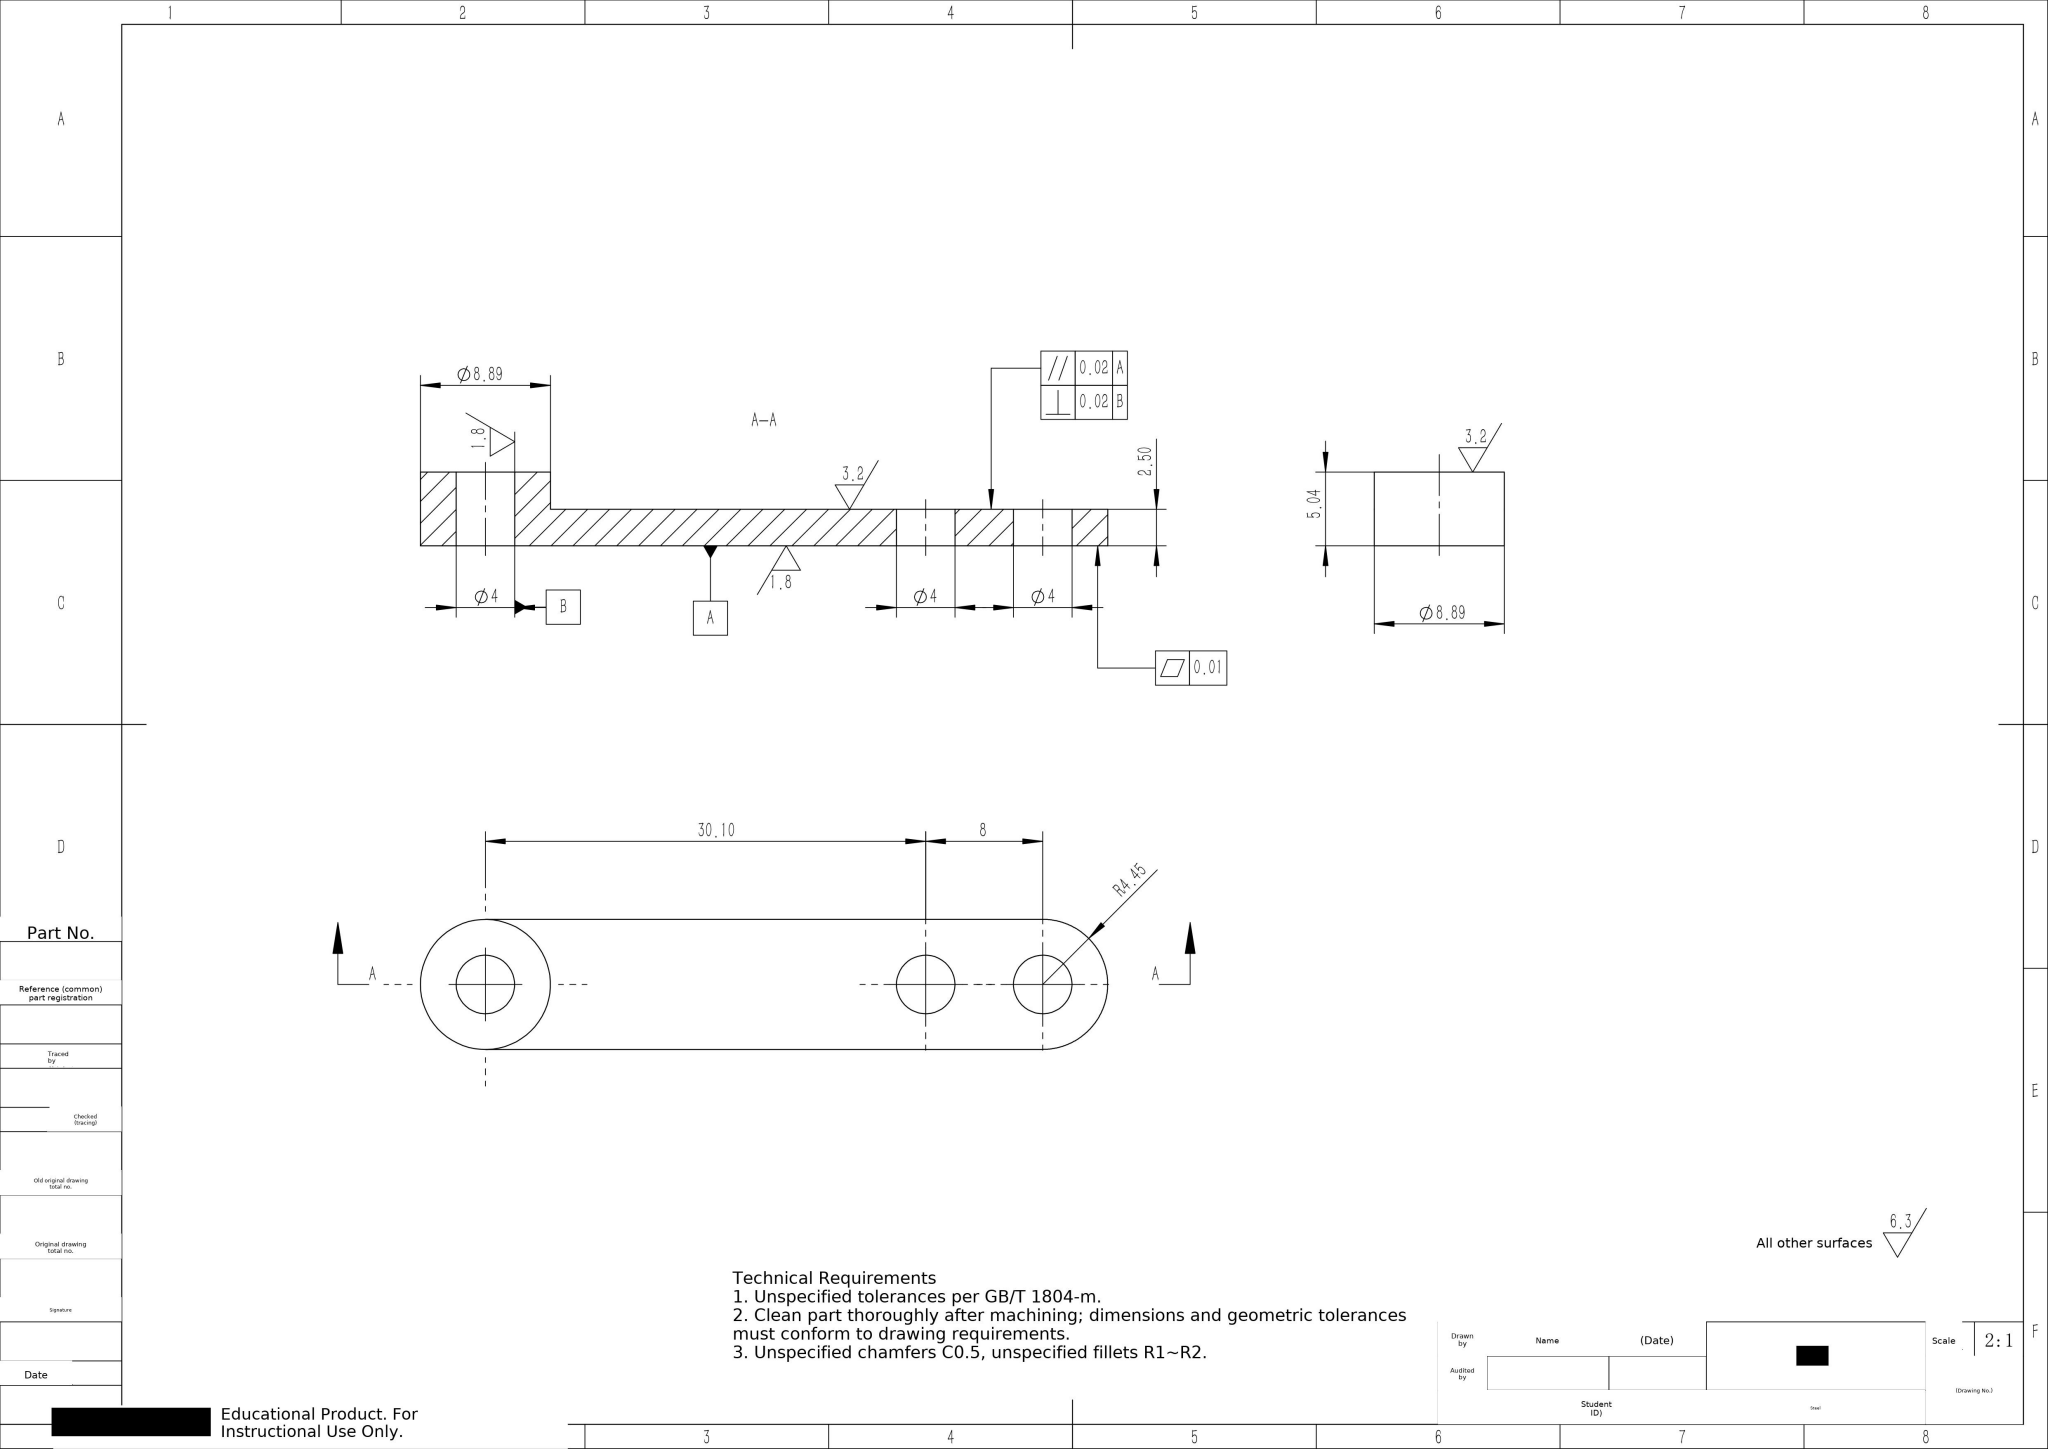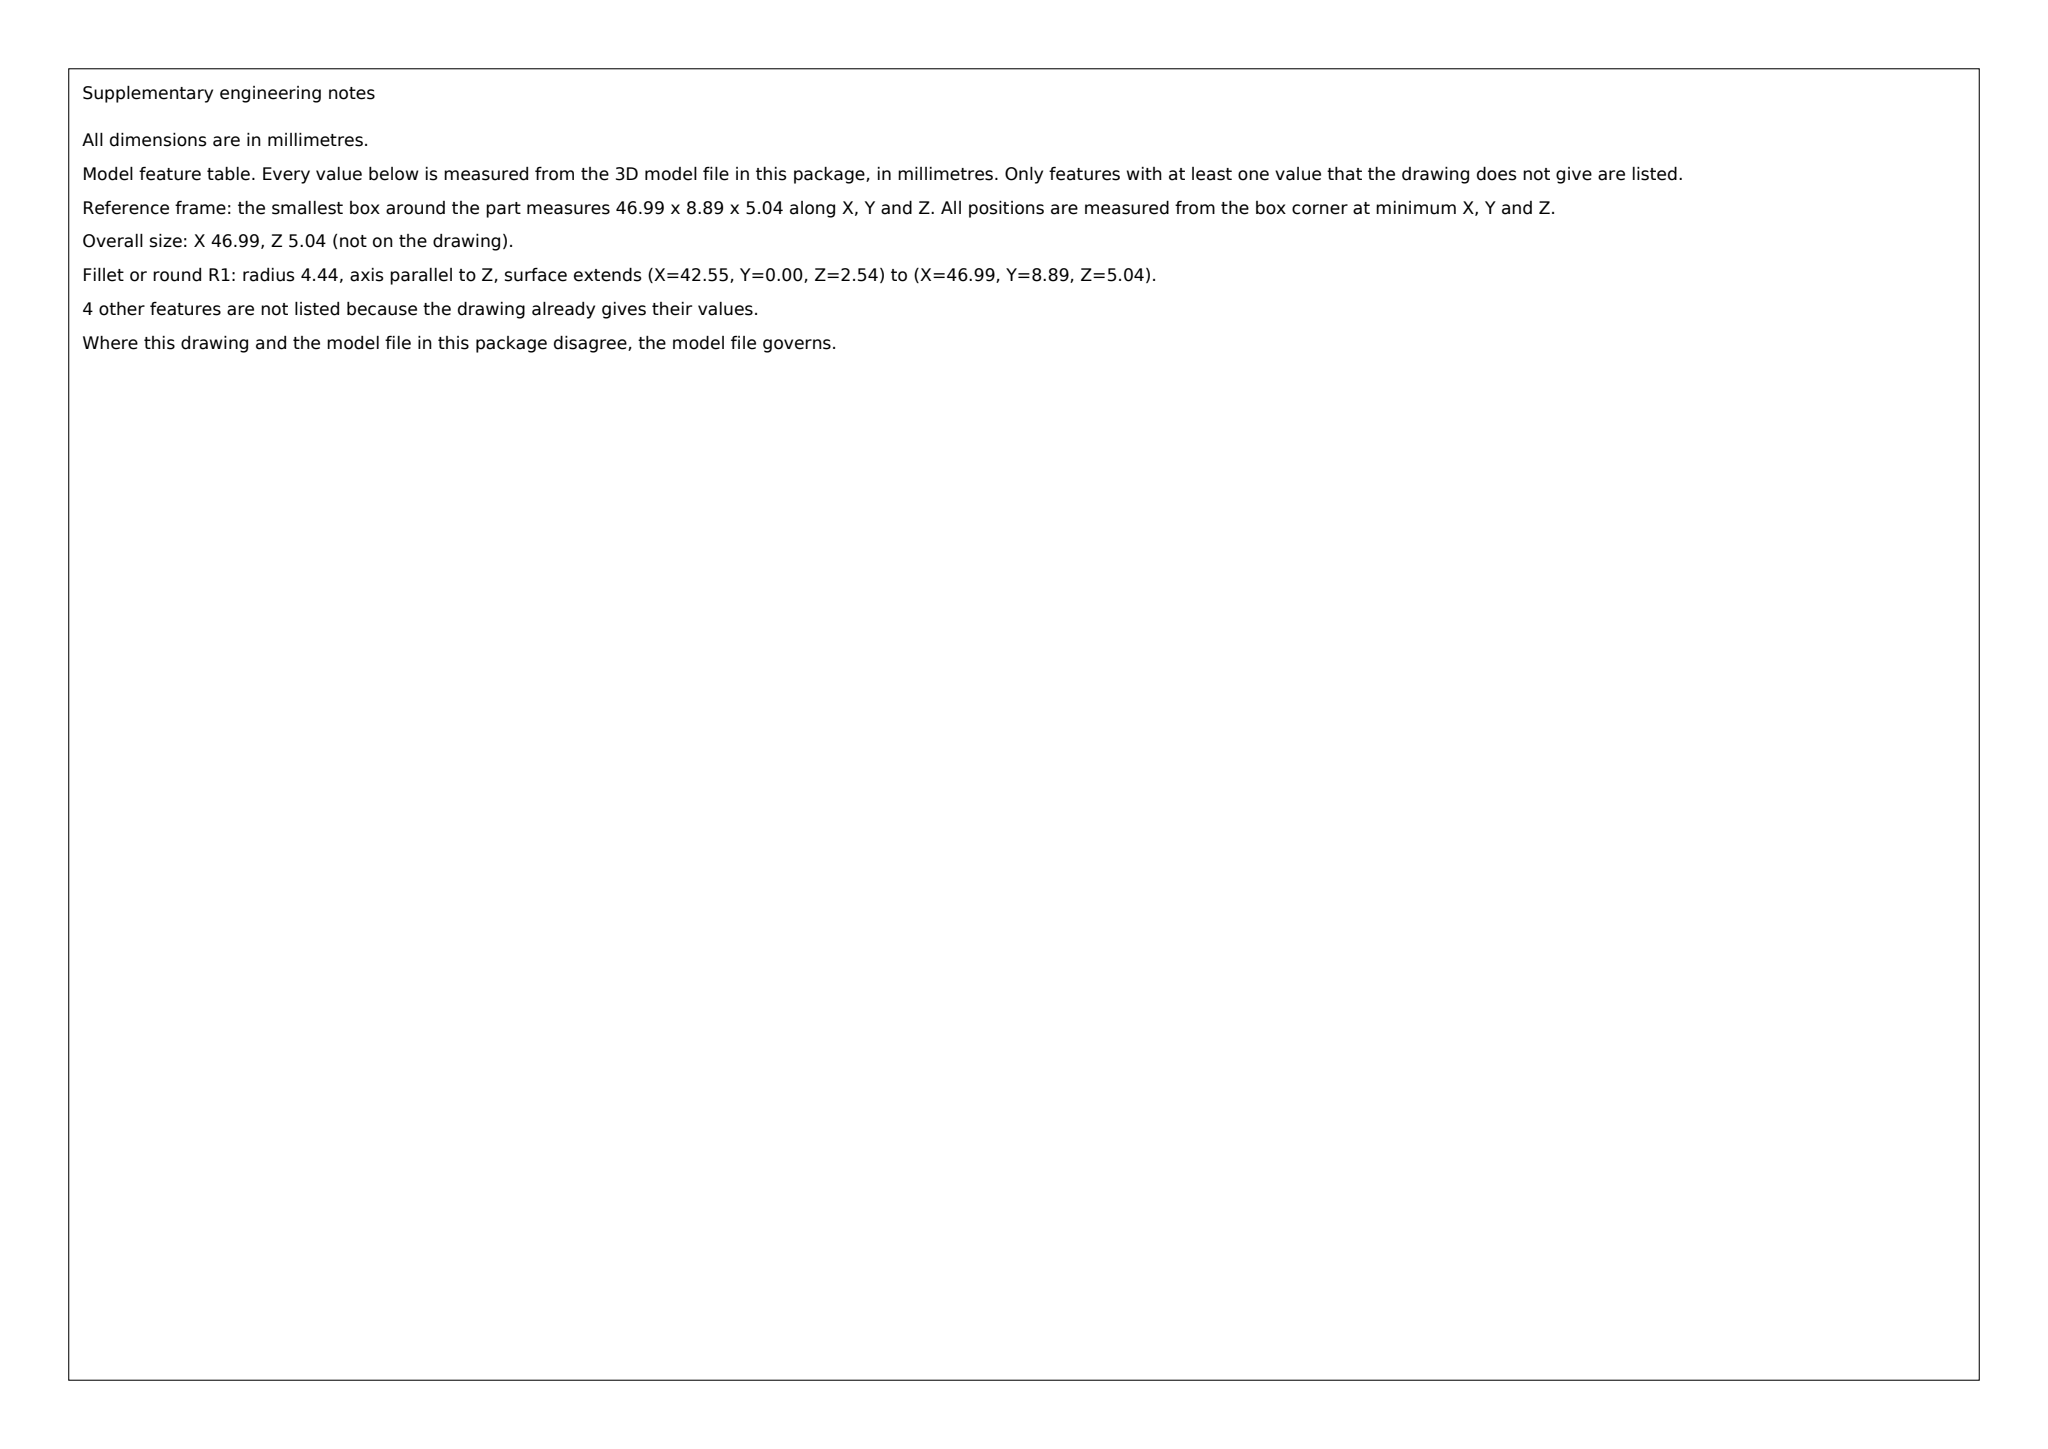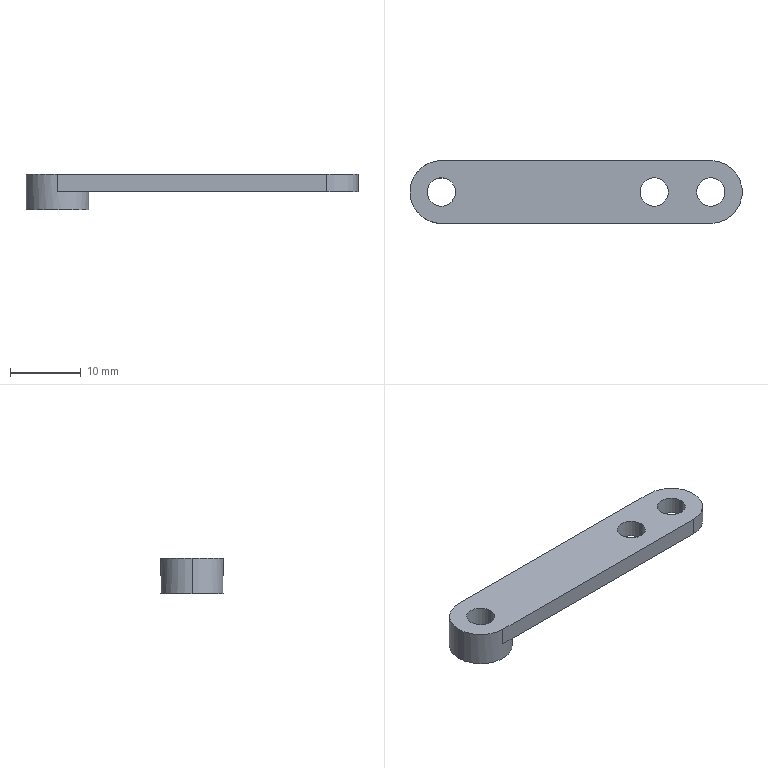Part | SolidWorks | mm | material Steel | 1 solid | 14 faces | box 46.99 x 8.89 x 5.04 mm | volume 1033 mm3 | cylinder 9 | plane 5 | commonest cylinder face diameters 4 x6 8.89 x3
build123d program:
from build123d import *

# Parameters (mm, degrees)
EXTRUDE1_DEPTH        = 2.5
SKETCH2_R             = 2
SKETCH2_R_2           = 1.5
CUT_EXTRUDE3_DEPTH    = 75.794
EXTRUDE2_START        = 2.54
SKETCH3_R             = 4.445
SKETCH3_R_2           = 1.587
EXTRUDE2_DEPTH        = 2.54
CROQUIS2_R            = 2
CORTAR_EXTRUIR2_DEPTH = 10


with BuildPart() as part:
    # Sketch1 → Extrude1 (new body)
    with BuildSketch(Plane.XY):
        with BuildLine():
            Line((-31.75, -8.255), (-69.85, -8.255))
            ThreePointArc((-69.85, -8.255), (-74.295, -3.81), (-69.85, 0.635))
            Line((-69.85, 0.635), (-31.75, 0.635))
            ThreePointArc((-31.75, 0.635), (-27.305, -3.81), (-31.75, -8.255))
        make_face()
    extrude(amount=EXTRUDE1_DEPTH)

    # Sketch2 → Cut-Extrude3 (cut, through all)
    with BuildSketch(Plane.XY):
        with Locations((-31.75, -3.81)):
            Circle(SKETCH2_R)
        with Locations((-39.75, -3.81)):
            Circle(SKETCH2_R)
        with Locations((-69.85, -3.81)):
            Circle(SKETCH2_R_2)
    extrude(amount=CUT_EXTRUDE3_DEPTH, mode=Mode.SUBTRACT)

    # Sketch3 → Extrude2 (add)
    with BuildSketch(Plane(origin=(0, 0, 0), x_dir=(-1, 0, 0), z_dir=(0, 0, -1)).offset(EXTRUDE2_START)):
        with Locations((69.85, -3.81)):
            Circle(SKETCH3_R)
        with Locations((69.85, -3.81)):
            Circle(SKETCH3_R_2, mode=Mode.SUBTRACT)
    extrude(amount=-EXTRUDE2_DEPTH)

    # Croquis2 → Cortar-Extruir2 (cut)
    with BuildSketch(Plane(origin=(0, 0, -2.54), x_dir=(-1, 0, 0), z_dir=(0, 0, -1))):
        with Locations((69.85, -3.81)):
            Circle(CROQUIS2_R)
    extrude(amount=-CORTAR_EXTRUIR2_DEPTH, mode=Mode.SUBTRACT)


solid = part.part
STEP:
#1=CARTESIAN_POINT('',(-71.85,-3.81,2.5));
#2=VERTEX_POINT('',#1);
#3=CARTESIAN_POINT('',(-67.85,-3.81,2.5));
#4=VERTEX_POINT('',#3);
#5=CARTESIAN_POINT('',(-69.85,-3.81,2.5));
#6=DIRECTION('',(0.,0.,1.));
#7=DIRECTION('',(1.,0.,0.));
#8=AXIS2_PLACEMENT_3D('',#5,#6,#7);
#9=CIRCLE('',#8,2.);
#10=EDGE_CURVE('',#2,#4,#9,.T.);
#11=ORIENTED_EDGE('',*,*,#10,.T.);
#12=CARTESIAN_POINT('',(-67.85,-3.81,-2.54));
#13=VERTEX_POINT('',#12);
#14=CARTESIAN_POINT('',(-67.85,-3.81,7.46));
#15=DIRECTION('',(0.,0.,-1.));
#16=VECTOR('',#15,1000.);
#17=LINE('',#14,#16);
#18=EDGE_CURVE('',#4,#13,#17,.T.);
#19=ORIENTED_EDGE('',*,*,#18,.T.);
#20=CARTESIAN_POINT('',(-71.85,-3.81,-2.54));
#21=VERTEX_POINT('',#20);
#22=CARTESIAN_POINT('',(-69.85,-3.81,-2.54));
#23=DIRECTION('',(0.,0.,-1.));
#24=DIRECTION('',(-1.,0.,0.));
#25=AXIS2_PLACEMENT_3D('',#22,#23,#24);
#26=CIRCLE('',#25,2.);
#27=EDGE_CURVE('',#13,#21,#26,.T.);
#28=ORIENTED_EDGE('',*,*,#27,.T.);
#29=CARTESIAN_POINT('',(-71.85,-3.81,7.46));
#30=DIRECTION('',(0.,0.,-1.));
#31=VECTOR('',#30,1000.);
#32=LINE('',#29,#31);
#33=EDGE_CURVE('',#2,#21,#32,.T.);
#34=ORIENTED_EDGE('',*,*,#33,.F.);
#35=EDGE_LOOP('',(#11,#19,#28,#34));
#36=FACE_OUTER_BOUND('',#35,.T.);
#37=CARTESIAN_POINT('',(-69.85,-3.81,7.46));
#38=DIRECTION('',(0.,0.,-1.));
#39=DIRECTION('',(-1.,0.,0.));
#40=AXIS2_PLACEMENT_3D('',#37,#38,#39);
#41=CYLINDRICAL_SURFACE('',#40,2.);
#42=ADVANCED_FACE('',(#36),#41,.F.);
#43=CARTESIAN_POINT('',(-41.75,-3.81,2.5));
#44=VERTEX_POINT('',#43);
#45=CARTESIAN_POINT('',(-37.75,-3.81,2.5));
#46=VERTEX_POINT('',#45);
#47=CARTESIAN_POINT('',(-39.75,-3.81,2.5));
#48=DIRECTION('',(0.,0.,1.));
#49=DIRECTION('',(1.,0.,0.));
#50=AXIS2_PLACEMENT_3D('',#47,#48,#49);
#51=CIRCLE('',#50,2.);
#52=EDGE_CURVE('',#44,#46,#51,.T.);
#53=ORIENTED_EDGE('',*,*,#52,.T.);
#54=CARTESIAN_POINT('',(-37.75,-3.81,0.));
#55=VERTEX_POINT('',#54);
#56=CARTESIAN_POINT('',(-37.75,-3.81,2.5));
#57=DIRECTION('',(0.,0.,-1.));
#58=VECTOR('',#57,1000.);
#59=LINE('',#56,#58);
#60=EDGE_CURVE('',#46,#55,#59,.T.);
#61=ORIENTED_EDGE('',*,*,#60,.T.);
#62=CARTESIAN_POINT('',(-41.75,-3.81,0.));
#63=VERTEX_POINT('',#62);
#64=CARTESIAN_POINT('',(-39.75,-3.81,0.));
#65=DIRECTION('',(0.,0.,1.));
#66=DIRECTION('',(1.,0.,0.));
#67=AXIS2_PLACEMENT_3D('',#64,#65,#66);
#68=CIRCLE('',#67,2.);
#69=EDGE_CURVE('',#63,#55,#68,.T.);
#70=ORIENTED_EDGE('',*,*,#69,.F.);
#71=CARTESIAN_POINT('',(-41.75,-3.81,2.5));
#72=DIRECTION('',(0.,0.,-1.));
#73=VECTOR('',#72,1000.);
#74=LINE('',#71,#73);
#75=EDGE_CURVE('',#44,#63,#74,.T.);
#76=ORIENTED_EDGE('',*,*,#75,.F.);
#77=EDGE_LOOP('',(#53,#61,#70,#76));
#78=FACE_OUTER_BOUND('',#77,.T.);
#79=CARTESIAN_POINT('',(-39.75,-3.81,2.5));
#80=DIRECTION('',(0.,0.,-1.));
#81=DIRECTION('',(-1.,0.,0.));
#82=AXIS2_PLACEMENT_3D('',#79,#80,#81);
#83=CYLINDRICAL_SURFACE('',#82,2.);
#84=ADVANCED_FACE('',(#78),#83,.F.);
#85=CARTESIAN_POINT('',(-33.75,-3.81,2.5));
#86=VERTEX_POINT('',#85);
#87=CARTESIAN_POINT('',(-29.75,-3.81,2.5));
#88=VERTEX_POINT('',#87);
#89=CARTESIAN_POINT('',(-31.75,-3.81,2.5));
#90=DIRECTION('',(0.,0.,1.));
#91=DIRECTION('',(1.,0.,0.));
#92=AXIS2_PLACEMENT_3D('',#89,#90,#91);
#93=CIRCLE('',#92,2.);
#94=EDGE_CURVE('',#86,#88,#93,.T.);
#95=ORIENTED_EDGE('',*,*,#94,.T.);
#96=CARTESIAN_POINT('',(-29.75,-3.81,0.));
#97=VERTEX_POINT('',#96);
#98=CARTESIAN_POINT('',(-29.75,-3.81,2.5));
#99=DIRECTION('',(0.,0.,-1.));
#100=VECTOR('',#99,1000.);
#101=LINE('',#98,#100);
#102=EDGE_CURVE('',#88,#97,#101,.T.);
#103=ORIENTED_EDGE('',*,*,#102,.T.);
#104=CARTESIAN_POINT('',(-33.75,-3.81,0.));
#105=VERTEX_POINT('',#104);
#106=CARTESIAN_POINT('',(-31.75,-3.81,0.));
#107=DIRECTION('',(0.,0.,1.));
#108=DIRECTION('',(1.,0.,0.));
#109=AXIS2_PLACEMENT_3D('',#106,#107,#108);
#110=CIRCLE('',#109,2.);
#111=EDGE_CURVE('',#105,#97,#110,.T.);
#112=ORIENTED_EDGE('',*,*,#111,.F.);
#113=CARTESIAN_POINT('',(-33.75,-3.81,2.5));
#114=DIRECTION('',(0.,0.,-1.));
#115=VECTOR('',#114,1000.);
#116=LINE('',#113,#115);
#117=EDGE_CURVE('',#86,#105,#116,.T.);
#118=ORIENTED_EDGE('',*,*,#117,.F.);
#119=EDGE_LOOP('',(#95,#103,#112,#118));
#120=FACE_OUTER_BOUND('',#119,.T.);
#121=CARTESIAN_POINT('',(-31.75,-3.81,2.5));
#122=DIRECTION('',(0.,0.,-1.));
#123=DIRECTION('',(-1.,0.,0.));
#124=AXIS2_PLACEMENT_3D('',#121,#122,#123);
#125=CYLINDRICAL_SURFACE('',#124,2.);
#126=ADVANCED_FACE('',(#120),#125,.F.);
#127=CARTESIAN_POINT('',(-69.85,0.635,0.));
#128=VERTEX_POINT('',#127);
#129=CARTESIAN_POINT('',(-65.405,-3.81,0.));
#130=VERTEX_POINT('',#129);
#131=CARTESIAN_POINT('',(-69.85,-3.81,0.));
#132=DIRECTION('',(0.,0.,-1.));
#133=DIRECTION('',(-1.,0.,0.));
#134=AXIS2_PLACEMENT_3D('',#131,#132,#133);
#135=CIRCLE('',#134,4.445);
#136=EDGE_CURVE('',#128,#130,#135,.T.);
#137=ORIENTED_EDGE('',*,*,#136,.T.);
#138=CARTESIAN_POINT('',(-65.405,-3.81,-2.54));
#139=VERTEX_POINT('',#138);
#140=CARTESIAN_POINT('',(-65.405,-3.81,2.5));
#141=DIRECTION('',(0.,0.,-1.));
#142=VECTOR('',#141,1000.);
#143=LINE('',#140,#142);
#144=EDGE_CURVE('',#130,#139,#143,.T.);
#145=ORIENTED_EDGE('',*,*,#144,.T.);
#146=CARTESIAN_POINT('',(-74.295,-3.81,-2.54));
#147=VERTEX_POINT('',#146);
#148=CARTESIAN_POINT('',(-69.85,-3.81,-2.54));
#149=DIRECTION('',(0.,0.,-1.));
#150=DIRECTION('',(-1.,0.,0.));
#151=AXIS2_PLACEMENT_3D('',#148,#149,#150);
#152=CIRCLE('',#151,4.445);
#153=EDGE_CURVE('',#147,#139,#152,.T.);
#154=ORIENTED_EDGE('',*,*,#153,.F.);
#155=CARTESIAN_POINT('',(-74.295,-3.81,2.5));
#156=VERTEX_POINT('',#155);
#157=CARTESIAN_POINT('',(-74.295,-3.81,2.5));
#158=DIRECTION('',(0.,0.,-1.));
#159=VECTOR('',#158,1000.);
#160=LINE('',#157,#159);
#161=EDGE_CURVE('',#156,#147,#160,.T.);
#162=ORIENTED_EDGE('',*,*,#161,.F.);
#163=CARTESIAN_POINT('',(-69.85,0.635,2.5));
#164=VERTEX_POINT('',#163);
#165=CARTESIAN_POINT('',(-69.85,-3.81,2.5));
#166=DIRECTION('',(0.,0.,1.));
#167=DIRECTION('',(1.,0.,0.));
#168=AXIS2_PLACEMENT_3D('',#165,#166,#167);
#169=CIRCLE('',#168,4.445);
#170=EDGE_CURVE('',#164,#156,#169,.T.);
#171=ORIENTED_EDGE('',*,*,#170,.F.);
#172=CARTESIAN_POINT('',(-69.85,0.635,2.5));
#173=DIRECTION('',(0.,0.,-1.));
#174=VECTOR('',#173,1000.);
#175=LINE('',#172,#174);
#176=EDGE_CURVE('',#164,#128,#175,.T.);
#177=ORIENTED_EDGE('',*,*,#176,.T.);
#178=EDGE_LOOP('',(#137,#145,#154,#162,#171,#177));
#179=FACE_OUTER_BOUND('',#178,.T.);
#180=CARTESIAN_POINT('',(-69.85,-3.81,2.5));
#181=DIRECTION('',(0.,0.,-1.));
#182=DIRECTION('',(-1.,0.,0.));
#183=AXIS2_PLACEMENT_3D('',#180,#181,#182);
#184=CYLINDRICAL_SURFACE('',#183,4.445);
#185=ADVANCED_FACE('',(#179),#184,.T.);
#186=ORIENTED_EDGE('',*,*,#111,.T.);
#187=CARTESIAN_POINT('',(-31.75,-3.81,0.));
#188=DIRECTION('',(0.,0.,1.));
#189=DIRECTION('',(1.,0.,0.));
#190=AXIS2_PLACEMENT_3D('',#187,#188,#189);
#191=CIRCLE('',#190,2.);
#192=EDGE_CURVE('',#97,#105,#191,.T.);
#193=ORIENTED_EDGE('',*,*,#192,.T.);
#194=EDGE_LOOP('',(#186,#193));
#195=FACE_BOUND('',#194,.T.);
#196=ORIENTED_EDGE('',*,*,#69,.T.);
#197=CARTESIAN_POINT('',(-39.75,-3.81,0.));
#198=DIRECTION('',(0.,0.,1.));
#199=DIRECTION('',(1.,0.,0.));
#200=AXIS2_PLACEMENT_3D('',#197,#198,#199);
#201=CIRCLE('',#200,2.);
#202=EDGE_CURVE('',#55,#63,#201,.T.);
#203=ORIENTED_EDGE('',*,*,#202,.T.);
#204=EDGE_LOOP('',(#196,#203));
#205=FACE_BOUND('',#204,.T.);
#206=ORIENTED_EDGE('',*,*,#136,.F.);
#207=CARTESIAN_POINT('',(-31.75,0.635,0.));
#208=VERTEX_POINT('',#207);
#209=CARTESIAN_POINT('',(-31.75,0.635,0.));
#210=DIRECTION('',(-1.,0.,0.));
#211=VECTOR('',#210,1000.);
#212=LINE('',#209,#211);
#213=EDGE_CURVE('',#208,#128,#212,.T.);
#214=ORIENTED_EDGE('',*,*,#213,.F.);
#215=CARTESIAN_POINT('',(-31.75,-8.255,0.));
#216=VERTEX_POINT('',#215);
#217=CARTESIAN_POINT('',(-31.75,-3.81,0.));
#218=DIRECTION('',(0.,0.,1.));
#219=DIRECTION('',(1.,0.,0.));
#220=AXIS2_PLACEMENT_3D('',#217,#218,#219);
#221=CIRCLE('',#220,4.445);
#222=EDGE_CURVE('',#216,#208,#221,.T.);
#223=ORIENTED_EDGE('',*,*,#222,.F.);
#224=CARTESIAN_POINT('',(-69.85,-8.255,0.));
#225=VERTEX_POINT('',#224);
#226=CARTESIAN_POINT('',(-31.75,-8.255,0.));
#227=DIRECTION('',(1.,0.,0.));
#228=VECTOR('',#227,1000.);
#229=LINE('',#226,#228);
#230=EDGE_CURVE('',#225,#216,#229,.T.);
#231=ORIENTED_EDGE('',*,*,#230,.F.);
#232=CARTESIAN_POINT('',(-69.85,-3.81,0.));
#233=DIRECTION('',(0.,0.,-1.));
#234=DIRECTION('',(-1.,0.,0.));
#235=AXIS2_PLACEMENT_3D('',#232,#233,#234);
#236=CIRCLE('',#235,4.445);
#237=EDGE_CURVE('',#130,#225,#236,.T.);
#238=ORIENTED_EDGE('',*,*,#237,.F.);
#239=EDGE_LOOP('',(#206,#214,#223,#231,#238));
#240=FACE_OUTER_BOUND('',#239,.T.);
#241=CARTESIAN_POINT('',(-31.75,-3.81,0.));
#242=DIRECTION('',(0.,0.,1.));
#243=DIRECTION('',(1.,0.,0.));
#244=AXIS2_PLACEMENT_3D('',#241,#242,#243);
#245=PLANE('',#244);
#246=ADVANCED_FACE('',(#195,#205,#240),#245,.F.);
#247=ORIENTED_EDGE('',*,*,#10,.F.);
#248=CARTESIAN_POINT('',(-69.85,-3.81,2.5));
#249=DIRECTION('',(0.,0.,1.));
#250=DIRECTION('',(1.,0.,0.));
#251=AXIS2_PLACEMENT_3D('',#248,#249,#250);
#252=CIRCLE('',#251,2.);
#253=EDGE_CURVE('',#4,#2,#252,.T.);
#254=ORIENTED_EDGE('',*,*,#253,.F.);
#255=EDGE_LOOP('',(#247,#254));
#256=FACE_BOUND('',#255,.T.);
#257=ORIENTED_EDGE('',*,*,#52,.F.);
#258=CARTESIAN_POINT('',(-39.75,-3.81,2.5));
#259=DIRECTION('',(0.,0.,1.));
#260=DIRECTION('',(1.,0.,0.));
#261=AXIS2_PLACEMENT_3D('',#258,#259,#260);
#262=CIRCLE('',#261,2.);
#263=EDGE_CURVE('',#46,#44,#262,.T.);
#264=ORIENTED_EDGE('',*,*,#263,.F.);
#265=EDGE_LOOP('',(#257,#264));
#266=FACE_BOUND('',#265,.T.);
#267=CARTESIAN_POINT('',(-31.75,-8.255,2.5));
#268=VERTEX_POINT('',#267);
#269=CARTESIAN_POINT('',(-31.75,0.635,2.5));
#270=VERTEX_POINT('',#269);
#271=CARTESIAN_POINT('',(-31.75,-3.81,2.5));
#272=DIRECTION('',(0.,0.,1.));
#273=DIRECTION('',(1.,0.,0.));
#274=AXIS2_PLACEMENT_3D('',#271,#272,#273);
#275=CIRCLE('',#274,4.445);
#276=EDGE_CURVE('',#268,#270,#275,.T.);
#277=ORIENTED_EDGE('',*,*,#276,.T.);
#278=CARTESIAN_POINT('',(-31.75,0.635,2.5));
#279=DIRECTION('',(-1.,0.,0.));
#280=VECTOR('',#279,1000.);
#281=LINE('',#278,#280);
#282=EDGE_CURVE('',#270,#164,#281,.T.);
#283=ORIENTED_EDGE('',*,*,#282,.T.);
#284=ORIENTED_EDGE('',*,*,#170,.T.);
#285=CARTESIAN_POINT('',(-69.85,-8.255,2.5));
#286=VERTEX_POINT('',#285);
#287=CARTESIAN_POINT('',(-69.85,-3.81,2.5));
#288=DIRECTION('',(0.,0.,1.));
#289=DIRECTION('',(1.,0.,0.));
#290=AXIS2_PLACEMENT_3D('',#287,#288,#289);
#291=CIRCLE('',#290,4.445);
#292=EDGE_CURVE('',#156,#286,#291,.T.);
#293=ORIENTED_EDGE('',*,*,#292,.T.);
#294=CARTESIAN_POINT('',(-31.75,-8.255,2.5));
#295=DIRECTION('',(1.,0.,0.));
#296=VECTOR('',#295,1000.);
#297=LINE('',#294,#296);
#298=EDGE_CURVE('',#286,#268,#297,.T.);
#299=ORIENTED_EDGE('',*,*,#298,.T.);
#300=EDGE_LOOP('',(#277,#283,#284,#293,#299));
#301=FACE_OUTER_BOUND('',#300,.T.);
#302=ORIENTED_EDGE('',*,*,#94,.F.);
#303=CARTESIAN_POINT('',(-31.75,-3.81,2.5));
#304=DIRECTION('',(0.,0.,1.));
#305=DIRECTION('',(1.,0.,0.));
#306=AXIS2_PLACEMENT_3D('',#303,#304,#305);
#307=CIRCLE('',#306,2.);
#308=EDGE_CURVE('',#88,#86,#307,.T.);
#309=ORIENTED_EDGE('',*,*,#308,.F.);
#310=EDGE_LOOP('',(#302,#309));
#311=FACE_BOUND('',#310,.T.);
#312=CARTESIAN_POINT('',(-31.75,-3.81,2.5));
#313=DIRECTION('',(0.,0.,1.));
#314=DIRECTION('',(1.,0.,0.));
#315=AXIS2_PLACEMENT_3D('',#312,#313,#314);
#316=PLANE('',#315);
#317=ADVANCED_FACE('',(#256,#266,#301,#311),#316,.T.);
#318=ORIENTED_EDGE('',*,*,#222,.T.);
#319=CARTESIAN_POINT('',(-31.75,0.635,2.5));
#320=DIRECTION('',(0.,0.,-1.));
#321=VECTOR('',#320,1000.);
#322=LINE('',#319,#321);
#323=EDGE_CURVE('',#270,#208,#322,.T.);
#324=ORIENTED_EDGE('',*,*,#323,.F.);
#325=ORIENTED_EDGE('',*,*,#276,.F.);
#326=CARTESIAN_POINT('',(-31.75,-8.255,2.5));
#327=DIRECTION('',(0.,0.,-1.));
#328=VECTOR('',#327,1000.);
#329=LINE('',#326,#328);
#330=EDGE_CURVE('',#268,#216,#329,.T.);
#331=ORIENTED_EDGE('',*,*,#330,.T.);
#332=EDGE_LOOP('',(#318,#324,#325,#331));
#333=FACE_OUTER_BOUND('',#332,.T.);
#334=CARTESIAN_POINT('',(-31.75,-3.81,2.5));
#335=DIRECTION('',(0.,0.,-1.));
#336=DIRECTION('',(-1.,0.,0.));
#337=AXIS2_PLACEMENT_3D('',#334,#335,#336);
#338=CYLINDRICAL_SURFACE('',#337,4.445);
#339=ADVANCED_FACE('',(#333),#338,.T.);
#340=ORIENTED_EDGE('',*,*,#213,.T.);
#341=ORIENTED_EDGE('',*,*,#176,.F.);
#342=ORIENTED_EDGE('',*,*,#282,.F.);
#343=ORIENTED_EDGE('',*,*,#323,.T.);
#344=EDGE_LOOP('',(#340,#341,#342,#343));
#345=FACE_OUTER_BOUND('',#344,.T.);
#346=CARTESIAN_POINT('',(-31.75,0.635,2.5));
#347=DIRECTION('',(0.,-1.,0.));
#348=DIRECTION('',(0.,0.,-1.));
#349=AXIS2_PLACEMENT_3D('',#346,#347,#348);
#350=PLANE('',#349);
#351=ADVANCED_FACE('',(#345),#350,.F.);
#352=ORIENTED_EDGE('',*,*,#144,.F.);
#353=ORIENTED_EDGE('',*,*,#237,.T.);
#354=CARTESIAN_POINT('',(-69.85,-8.255,2.5));
#355=DIRECTION('',(0.,0.,-1.));
#356=VECTOR('',#355,1000.);
#357=LINE('',#354,#356);
#358=EDGE_CURVE('',#286,#225,#357,.T.);
#359=ORIENTED_EDGE('',*,*,#358,.F.);
#360=ORIENTED_EDGE('',*,*,#292,.F.);
#361=ORIENTED_EDGE('',*,*,#161,.T.);
#362=CARTESIAN_POINT('',(-69.85,-3.81,-2.54));
#363=DIRECTION('',(0.,0.,-1.));
#364=DIRECTION('',(-1.,0.,0.));
#365=AXIS2_PLACEMENT_3D('',#362,#363,#364);
#366=CIRCLE('',#365,4.445);
#367=EDGE_CURVE('',#139,#147,#366,.T.);
#368=ORIENTED_EDGE('',*,*,#367,.F.);
#369=EDGE_LOOP('',(#352,#353,#359,#360,#361,#368));
#370=FACE_OUTER_BOUND('',#369,.T.);
#371=CARTESIAN_POINT('',(-69.85,-3.81,2.5));
#372=DIRECTION('',(0.,0.,-1.));
#373=DIRECTION('',(-1.,0.,0.));
#374=AXIS2_PLACEMENT_3D('',#371,#372,#373);
#375=CYLINDRICAL_SURFACE('',#374,4.445);
#376=ADVANCED_FACE('',(#370),#375,.T.);
#377=ORIENTED_EDGE('',*,*,#230,.T.);
#378=ORIENTED_EDGE('',*,*,#330,.F.);
#379=ORIENTED_EDGE('',*,*,#298,.F.);
#380=ORIENTED_EDGE('',*,*,#358,.T.);
#381=EDGE_LOOP('',(#377,#378,#379,#380));
#382=FACE_OUTER_BOUND('',#381,.T.);
#383=CARTESIAN_POINT('',(-31.75,-8.255,2.5));
#384=DIRECTION('',(0.,1.,0.));
#385=DIRECTION('',(0.,0.,1.));
#386=AXIS2_PLACEMENT_3D('',#383,#384,#385);
#387=PLANE('',#386);
#388=ADVANCED_FACE('',(#382),#387,.F.);
#389=ORIENTED_EDGE('',*,*,#102,.F.);
#390=ORIENTED_EDGE('',*,*,#308,.T.);
#391=ORIENTED_EDGE('',*,*,#117,.T.);
#392=ORIENTED_EDGE('',*,*,#192,.F.);
#393=EDGE_LOOP('',(#389,#390,#391,#392));
#394=FACE_OUTER_BOUND('',#393,.T.);
#395=CARTESIAN_POINT('',(-31.75,-3.81,2.5));
#396=DIRECTION('',(0.,0.,-1.));
#397=DIRECTION('',(-1.,0.,0.));
#398=AXIS2_PLACEMENT_3D('',#395,#396,#397);
#399=CYLINDRICAL_SURFACE('',#398,2.);
#400=ADVANCED_FACE('',(#394),#399,.F.);
#401=ORIENTED_EDGE('',*,*,#60,.F.);
#402=ORIENTED_EDGE('',*,*,#263,.T.);
#403=ORIENTED_EDGE('',*,*,#75,.T.);
#404=ORIENTED_EDGE('',*,*,#202,.F.);
#405=EDGE_LOOP('',(#401,#402,#403,#404));
#406=FACE_OUTER_BOUND('',#405,.T.);
#407=CARTESIAN_POINT('',(-39.75,-3.81,2.5));
#408=DIRECTION('',(0.,0.,-1.));
#409=DIRECTION('',(-1.,0.,0.));
#410=AXIS2_PLACEMENT_3D('',#407,#408,#409);
#411=CYLINDRICAL_SURFACE('',#410,2.);
#412=ADVANCED_FACE('',(#406),#411,.F.);
#413=CARTESIAN_POINT('',(-69.85,-3.81,-2.54));
#414=DIRECTION('',(0.,0.,-1.));
#415=DIRECTION('',(-1.,0.,0.));
#416=AXIS2_PLACEMENT_3D('',#413,#414,#415);
#417=CIRCLE('',#416,2.);
#418=EDGE_CURVE('',#21,#13,#417,.T.);
#419=ORIENTED_EDGE('',*,*,#418,.F.);
#420=ORIENTED_EDGE('',*,*,#27,.F.);
#421=EDGE_LOOP('',(#419,#420));
#422=FACE_BOUND('',#421,.T.);
#423=ORIENTED_EDGE('',*,*,#153,.T.);
#424=ORIENTED_EDGE('',*,*,#367,.T.);
#425=EDGE_LOOP('',(#423,#424));
#426=FACE_OUTER_BOUND('',#425,.T.);
#427=CARTESIAN_POINT('',(-69.85,-3.81,-2.54));
#428=DIRECTION('',(0.,0.,-1.));
#429=DIRECTION('',(-1.,0.,0.));
#430=AXIS2_PLACEMENT_3D('',#427,#428,#429);
#431=PLANE('',#430);
#432=ADVANCED_FACE('',(#422,#426),#431,.T.);
#433=ORIENTED_EDGE('',*,*,#18,.F.);
#434=ORIENTED_EDGE('',*,*,#253,.T.);
#435=ORIENTED_EDGE('',*,*,#33,.T.);
#436=ORIENTED_EDGE('',*,*,#418,.T.);
#437=EDGE_LOOP('',(#433,#434,#435,#436));
#438=FACE_OUTER_BOUND('',#437,.T.);
#439=CARTESIAN_POINT('',(-69.85,-3.81,7.46));
#440=DIRECTION('',(0.,0.,-1.));
#441=DIRECTION('',(-1.,0.,0.));
#442=AXIS2_PLACEMENT_3D('',#439,#440,#441);
#443=CYLINDRICAL_SURFACE('',#442,2.);
#444=ADVANCED_FACE('',(#438),#443,.F.);
#445=CLOSED_SHELL('',(#42,#84,#126,#185,#246,#317,#339,#351,#376,#388,#400,#412,#432,#444));
#446=MANIFOLD_SOLID_BREP('',#445);
#447=CARTESIAN_POINT('',(0.,0.,0.));
#448=DIRECTION('',(0.,0.,1.));
#449=DIRECTION('',(1.,0.,0.));
#450=AXIS2_PLACEMENT_3D('',#447,#448,#449);
#451=(LENGTH_UNIT()NAMED_UNIT(*)SI_UNIT(.MILLI.,.METRE.));
#452=UNCERTAINTY_MEASURE_WITH_UNIT(LENGTH_MEASURE(0.00001),#451,'','');
#453=(NAMED_UNIT(*)PLANE_ANGLE_UNIT()SI_UNIT($,.RADIAN.));
#454=(NAMED_UNIT(*)SI_UNIT($,.STERADIAN.)SOLID_ANGLE_UNIT());
#455=(GEOMETRIC_REPRESENTATION_CONTEXT(3)GLOBAL_UNCERTAINTY_ASSIGNED_CONTEXT((#452))GLOBAL_UNIT_ASSIGNED_CONTEXT((#451,#453,#454))REPRESENTATION_CONTEXT('',''));
#456=ADVANCED_BREP_SHAPE_REPRESENTATION('',(#446,#450),#455);